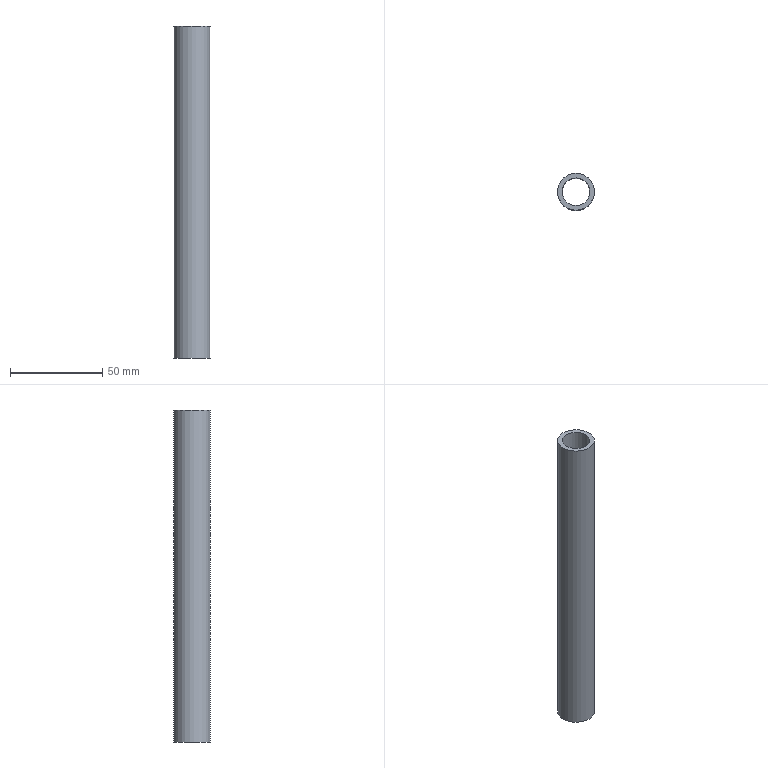Component | NX | SUPPORT_ROD_1 | 1 solid | 4 faces | box 20 x 20 x 180 mm | volume 24740 mm3 | plane 2 | cylinder 2 | commonest cylinder face diameters 20 x1 15 x1
STEP:
#1=CARTESIAN_POINT('',(0.,0.,0.));
#2=DIRECTION('',(0.,0.,1.));
#3=DIRECTION('',(1.,0.,0.));
#4=AXIS2_PLACEMENT_3D('',#1,#2,#3);
#5=CARTESIAN_POINT('',(35.864,19.626,960.));
#6=VERTEX_POINT('',#5);
#7=CARTESIAN_POINT('',(35.864,12.126,960.));
#8=DIRECTION('',(0.,0.,-1.));
#9=DIRECTION('',(0.,1.,0.));
#10=AXIS2_PLACEMENT_3D('',#7,#8,#9);
#11=CIRCLE('',#10,7.5);
#12=CARTESIAN_POINT('',(35.864,12.126,960.));
#13=DIRECTION('',(0.,0.,1.));
#14=DIRECTION('',(0.,-1.,0.));
#15=AXIS2_PLACEMENT_3D('',#12,#13,#14);
#16=PLANE('',#15);
#17=CARTESIAN_POINT('',(-7.5,0.));
#18=CARTESIAN_POINT('',(-7.5,12.99));
#19=CARTESIAN_POINT('',(3.75,6.495));
#20=CARTESIAN_POINT('',(15.,0.));
#21=CARTESIAN_POINT('',(3.75,-6.495));
#22=CARTESIAN_POINT('',(-7.5,-12.99));
#23=CARTESIAN_POINT('',(-7.5,0.));
#24=(BOUNDED_CURVE()B_SPLINE_CURVE(2,(#17,#18,#19,#20,#21,#22,#23),.UNSPECIFIED.,.T.,.F.)B_SPLINE_CURVE_WITH_KNOTS((1,2,2,2,2,1),(-2.094,0.,2.094,4.189,6.283,8.378),.UNSPECIFIED.)CURVE()GEOMETRIC_REPRESENTATION_ITEM()RATIONAL_B_SPLINE_CURVE((1.,0.5,1.,0.5,1.,0.5,1.))REPRESENTATION_ITEM(''));
#25=(GEOMETRIC_REPRESENTATION_CONTEXT(2)PARAMETRIC_REPRESENTATION_CONTEXT()REPRESENTATION_CONTEXT('',''));
#26=DEFINITIONAL_REPRESENTATION('',(#24),#25);
#27=PCURVE('',#16,#26);
#28=CARTESIAN_POINT('',(35.864,12.126,960.));
#29=DIRECTION('',(0.,0.,-1.));
#30=DIRECTION('',(0.,1.,0.));
#31=AXIS2_PLACEMENT_3D('',#28,#29,#30);
#32=CYLINDRICAL_SURFACE('',#31,7.5);
#33=CARTESIAN_POINT('',(0.,0.));
#34=DIRECTION('',(1.,0.));
#35=VECTOR('',#34,1.);
#36=LINE('',#33,#35);
#37=(GEOMETRIC_REPRESENTATION_CONTEXT(2)PARAMETRIC_REPRESENTATION_CONTEXT()REPRESENTATION_CONTEXT('',''));
#38=DEFINITIONAL_REPRESENTATION('',(#36),#37);
#39=PCURVE('',#32,#38);
#40=SURFACE_CURVE('',#11,(#27,#39),.PCURVE_S1.);
#41=EDGE_CURVE('',#6,#6,#40,.T.);
#42=ORIENTED_EDGE('',*,*,#41,.T.);
#43=EDGE_LOOP('',(#42));
#44=FACE_BOUND('',#43,.T.);
#45=CARTESIAN_POINT('',(35.864,2.126,960.));
#46=VERTEX_POINT('',#45);
#47=CARTESIAN_POINT('',(35.864,12.126,960.));
#48=DIRECTION('',(0.,0.,-1.));
#49=DIRECTION('',(0.,-1.,0.));
#50=AXIS2_PLACEMENT_3D('',#47,#48,#49);
#51=CIRCLE('',#50,10.);
#52=CARTESIAN_POINT('',(10.,0.));
#53=CARTESIAN_POINT('',(10.,-17.321));
#54=CARTESIAN_POINT('',(-5.,-8.66));
#55=CARTESIAN_POINT('',(-20.,-0.));
#56=CARTESIAN_POINT('',(-5.,8.66));
#57=CARTESIAN_POINT('',(10.,17.321));
#58=CARTESIAN_POINT('',(10.,0.));
#59=(BOUNDED_CURVE()B_SPLINE_CURVE(2,(#52,#53,#54,#55,#56,#57,#58),.UNSPECIFIED.,.T.,.F.)B_SPLINE_CURVE_WITH_KNOTS((1,2,2,2,2,1),(-2.094,0.,2.094,4.189,6.283,8.378),.UNSPECIFIED.)CURVE()GEOMETRIC_REPRESENTATION_ITEM()RATIONAL_B_SPLINE_CURVE((1.,0.5,1.,0.5,1.,0.5,1.))REPRESENTATION_ITEM(''));
#60=(GEOMETRIC_REPRESENTATION_CONTEXT(2)PARAMETRIC_REPRESENTATION_CONTEXT()REPRESENTATION_CONTEXT('',''));
#61=DEFINITIONAL_REPRESENTATION('',(#59),#60);
#62=PCURVE('',#16,#61);
#63=CARTESIAN_POINT('',(35.864,12.126,780.));
#64=DIRECTION('',(0.,0.,1.));
#65=DIRECTION('',(0.,-1.,0.));
#66=AXIS2_PLACEMENT_3D('',#63,#64,#65);
#67=CYLINDRICAL_SURFACE('',#66,10.);
#68=CARTESIAN_POINT('',(6.283,180.));
#69=DIRECTION('',(-1.,0.));
#70=VECTOR('',#69,1.);
#71=LINE('',#68,#70);
#72=(GEOMETRIC_REPRESENTATION_CONTEXT(2)PARAMETRIC_REPRESENTATION_CONTEXT()REPRESENTATION_CONTEXT('',''));
#73=DEFINITIONAL_REPRESENTATION('',(#71),#72);
#74=PCURVE('',#67,#73);
#75=SURFACE_CURVE('',#51,(#62,#74),.PCURVE_S1.);
#76=EDGE_CURVE('',#46,#46,#75,.T.);
#77=ORIENTED_EDGE('',*,*,#76,.F.);
#78=EDGE_LOOP('',(#77));
#79=FACE_BOUND('',#78,.T.);
#80=ADVANCED_FACE('',(#44,#79),#16,.T.);
#81=CARTESIAN_POINT('',(35.864,19.626,780.));
#82=VERTEX_POINT('',#81);
#83=CARTESIAN_POINT('',(35.864,12.126,780.));
#84=DIRECTION('',(0.,0.,-1.));
#85=DIRECTION('',(0.,1.,0.));
#86=AXIS2_PLACEMENT_3D('',#83,#84,#85);
#87=CIRCLE('',#86,7.5);
#88=CARTESIAN_POINT('',(35.864,12.126,780.));
#89=DIRECTION('',(0.,0.,-1.));
#90=DIRECTION('',(0.,1.,0.));
#91=AXIS2_PLACEMENT_3D('',#88,#89,#90);
#92=PLANE('',#91);
#93=CARTESIAN_POINT('',(0.,0.));
#94=DIRECTION('',(1.,0.));
#95=AXIS2_PLACEMENT_2D('',#93,#94);
#96=CIRCLE('',#95,7.5);
#97=(GEOMETRIC_REPRESENTATION_CONTEXT(2)PARAMETRIC_REPRESENTATION_CONTEXT()REPRESENTATION_CONTEXT('',''));
#98=DEFINITIONAL_REPRESENTATION('',(#96),#97);
#99=PCURVE('',#92,#98);
#100=CARTESIAN_POINT('',(0.,180.));
#101=DIRECTION('',(1.,0.));
#102=VECTOR('',#101,1.);
#103=LINE('',#100,#102);
#104=(GEOMETRIC_REPRESENTATION_CONTEXT(2)PARAMETRIC_REPRESENTATION_CONTEXT()REPRESENTATION_CONTEXT('',''));
#105=DEFINITIONAL_REPRESENTATION('',(#103),#104);
#106=PCURVE('',#32,#105);
#107=SURFACE_CURVE('',#87,(#99,#106),.PCURVE_S1.);
#108=EDGE_CURVE('',#82,#82,#107,.T.);
#109=ORIENTED_EDGE('',*,*,#108,.F.);
#110=EDGE_LOOP('',(#109));
#111=FACE_BOUND('',#110,.T.);
#112=CARTESIAN_POINT('',(35.864,2.126,780.));
#113=VERTEX_POINT('',#112);
#114=CARTESIAN_POINT('',(35.864,12.126,780.));
#115=DIRECTION('',(0.,0.,1.));
#116=DIRECTION('',(0.,-1.,0.));
#117=AXIS2_PLACEMENT_3D('',#114,#115,#116);
#118=CIRCLE('',#117,10.);
#119=CARTESIAN_POINT('',(-10.,0.));
#120=CARTESIAN_POINT('',(-10.,17.321));
#121=CARTESIAN_POINT('',(5.,8.66));
#122=CARTESIAN_POINT('',(20.,0.));
#123=CARTESIAN_POINT('',(5.,-8.66));
#124=CARTESIAN_POINT('',(-10.,-17.321));
#125=CARTESIAN_POINT('',(-10.,0.));
#126=(BOUNDED_CURVE()B_SPLINE_CURVE(2,(#119,#120,#121,#122,#123,#124,#125),.UNSPECIFIED.,.T.,.F.)B_SPLINE_CURVE_WITH_KNOTS((1,2,2,2,2,1),(-2.094,0.,2.094,4.189,6.283,8.378),.UNSPECIFIED.)CURVE()GEOMETRIC_REPRESENTATION_ITEM()RATIONAL_B_SPLINE_CURVE((1.,0.5,1.,0.5,1.,0.5,1.))REPRESENTATION_ITEM(''));
#127=(GEOMETRIC_REPRESENTATION_CONTEXT(2)PARAMETRIC_REPRESENTATION_CONTEXT()REPRESENTATION_CONTEXT('',''));
#128=DEFINITIONAL_REPRESENTATION('',(#126),#127);
#129=PCURVE('',#92,#128);
#130=CARTESIAN_POINT('',(0.,0.));
#131=DIRECTION('',(1.,0.));
#132=VECTOR('',#131,1.);
#133=LINE('',#130,#132);
#134=(GEOMETRIC_REPRESENTATION_CONTEXT(2)PARAMETRIC_REPRESENTATION_CONTEXT()REPRESENTATION_CONTEXT('',''));
#135=DEFINITIONAL_REPRESENTATION('',(#133),#134);
#136=PCURVE('',#67,#135);
#137=SURFACE_CURVE('',#118,(#129,#136),.PCURVE_S1.);
#138=EDGE_CURVE('',#113,#113,#137,.T.);
#139=ORIENTED_EDGE('',*,*,#138,.F.);
#140=EDGE_LOOP('',(#139));
#141=FACE_BOUND('',#140,.T.);
#142=ADVANCED_FACE('',(#111,#141),#92,.T.);
#143=ORIENTED_EDGE('',*,*,#76,.T.);
#144=CARTESIAN_POINT('',(35.864,2.126,780.));
#145=CARTESIAN_POINT('',(35.864,2.126,960.));
#146=B_SPLINE_CURVE_WITH_KNOTS('',1,(#144,#145),.UNSPECIFIED.,.F.,.F.,(2,2),(0.,180.),.PIECEWISE_BEZIER_KNOTS.);
#147=CARTESIAN_POINT('',(0.,0.));
#148=DIRECTION('',(0.,1.));
#149=VECTOR('',#148,1.);
#150=LINE('',#147,#149);
#151=(GEOMETRIC_REPRESENTATION_CONTEXT(2)PARAMETRIC_REPRESENTATION_CONTEXT()REPRESENTATION_CONTEXT('',''));
#152=DEFINITIONAL_REPRESENTATION('',(#150),#151);
#153=PCURVE('',#67,#152);
#154=CARTESIAN_POINT('',(6.283,0.));
#155=DIRECTION('',(0.,1.));
#156=VECTOR('',#155,1.);
#157=LINE('',#154,#156);
#158=(GEOMETRIC_REPRESENTATION_CONTEXT(2)PARAMETRIC_REPRESENTATION_CONTEXT()REPRESENTATION_CONTEXT('',''));
#159=DEFINITIONAL_REPRESENTATION('',(#157),#158);
#160=PCURVE('',#67,#159);
#161=SEAM_CURVE('',#146,(#153,#160),.PCURVE_S1.);
#162=EDGE_CURVE('',#113,#46,#161,.T.);
#163=ORIENTED_EDGE('',*,*,#162,.F.);
#164=ORIENTED_EDGE('',*,*,#138,.T.);
#165=ORIENTED_EDGE('',*,*,#162,.T.);
#166=EDGE_LOOP('',(#143,#163,#164,#165));
#167=FACE_BOUND('',#166,.T.);
#168=ADVANCED_FACE('',(#167),#67,.T.);
#169=ORIENTED_EDGE('',*,*,#108,.F.);
#170=CARTESIAN_POINT('',(35.864,19.626,960.));
#171=CARTESIAN_POINT('',(35.864,19.626,780.));
#172=B_SPLINE_CURVE_WITH_KNOTS('',1,(#170,#171),.UNSPECIFIED.,.F.,.F.,(2,2),(0.,180.),.PIECEWISE_BEZIER_KNOTS.);
#173=CARTESIAN_POINT('',(0.,0.));
#174=DIRECTION('',(0.,1.));
#175=VECTOR('',#174,1.);
#176=LINE('',#173,#175);
#177=(GEOMETRIC_REPRESENTATION_CONTEXT(2)PARAMETRIC_REPRESENTATION_CONTEXT()REPRESENTATION_CONTEXT('',''));
#178=DEFINITIONAL_REPRESENTATION('',(#176),#177);
#179=PCURVE('',#32,#178);
#180=CARTESIAN_POINT('',(6.283,0.));
#181=DIRECTION('',(0.,1.));
#182=VECTOR('',#181,1.);
#183=LINE('',#180,#182);
#184=(GEOMETRIC_REPRESENTATION_CONTEXT(2)PARAMETRIC_REPRESENTATION_CONTEXT()REPRESENTATION_CONTEXT('',''));
#185=DEFINITIONAL_REPRESENTATION('',(#183),#184);
#186=PCURVE('',#32,#185);
#187=SEAM_CURVE('',#172,(#179,#186),.PCURVE_S1.);
#188=EDGE_CURVE('',#6,#82,#187,.T.);
#189=ORIENTED_EDGE('',*,*,#188,.F.);
#190=ORIENTED_EDGE('',*,*,#41,.T.);
#191=ORIENTED_EDGE('',*,*,#188,.T.);
#192=EDGE_LOOP('',(#169,#189,#190,#191));
#193=FACE_BOUND('',#192,.F.);
#194=ADVANCED_FACE('',(#193),#32,.F.);
#195=CLOSED_SHELL('',(#80,#142,#168,#194));
#196=MANIFOLD_SOLID_BREP('',#195);
#197=(LENGTH_UNIT()NAMED_UNIT(*)SI_UNIT(.MILLI.,.METRE.));
#198=UNCERTAINTY_MEASURE_WITH_UNIT(LENGTH_MEASURE(0.00001),#197,'','');
#199=(NAMED_UNIT(*)PLANE_ANGLE_UNIT()SI_UNIT($,.RADIAN.));
#200=(NAMED_UNIT(*)SI_UNIT($,.STERADIAN.)SOLID_ANGLE_UNIT());
#201=(GEOMETRIC_REPRESENTATION_CONTEXT(3)GLOBAL_UNCERTAINTY_ASSIGNED_CONTEXT((#198))GLOBAL_UNIT_ASSIGNED_CONTEXT((#197,#199,#200))REPRESENTATION_CONTEXT('',''));
#202=ADVANCED_BREP_SHAPE_REPRESENTATION('',(#4,#196),#201);